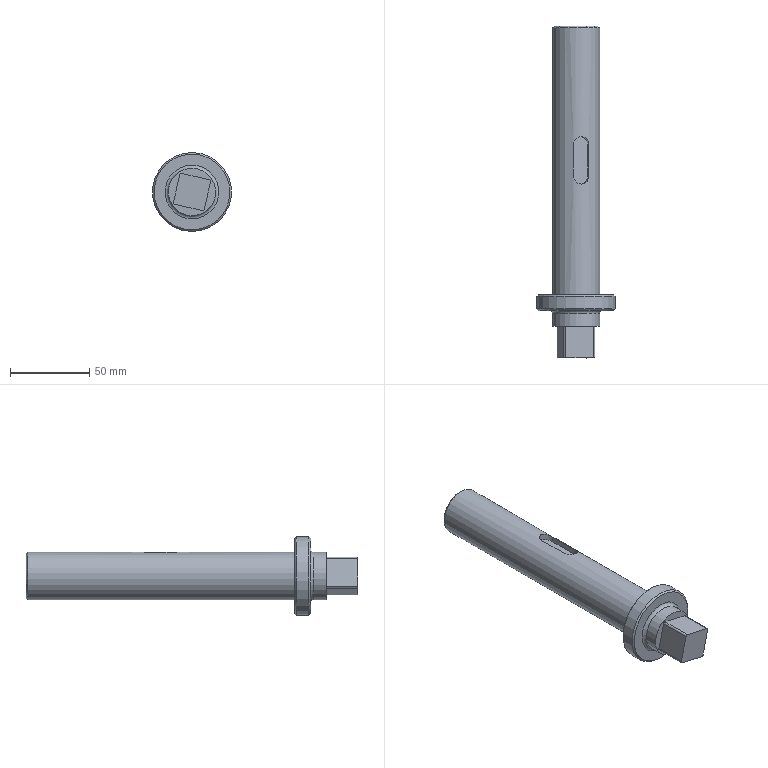Component | NX | SPINDLE | 1 solid | 25 faces | volume 153694 mm3 | plane 12 | cylinder 9 | cone 3 | torus 1 | commonest cylinder face diameters 2 x4 30 x2 10 x2 50 x1